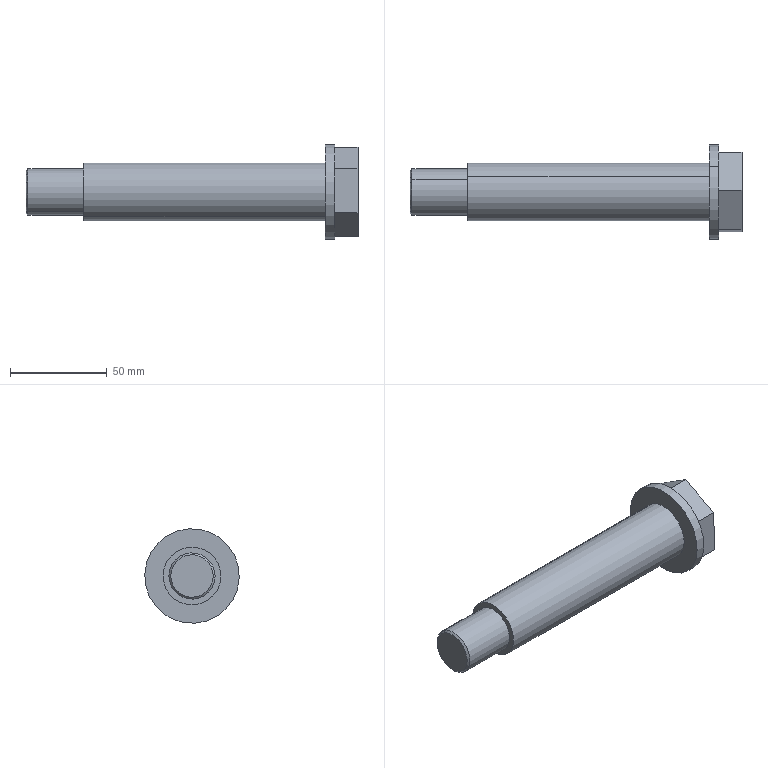Component | SolidWorks | SeedingAssemblyA-1_SeedingAxis-1 | 1 solid | 19 faces | box 172 x 49 x 49 mm | volume 127949 mm3 | plane 11 | cylinder 6 | cone 2 | commonest cylinder face diameters 24 x2 49 x2 30 x2
STEP:
#1=COLOUR_RGB('',0.7922,0.8196,0.9333);
#2=FILL_AREA_STYLE_COLOUR('',#1);
#3=FILL_AREA_STYLE('',(#2));
#4=SURFACE_STYLE_FILL_AREA(#3);
#5=SURFACE_SIDE_STYLE('',(#4));
#6=SURFACE_STYLE_USAGE(.BOTH.,#5);
#7=PRESENTATION_STYLE_ASSIGNMENT((#6));
#8=CARTESIAN_POINT('',(-0.3631,-3.902,-9.563));
#9=VERTEX_POINT('',#8);
#10=CARTESIAN_POINT('',(-0.3631,-4.366,-10.294));
#11=VERTEX_POINT('',#10);
#12=CARTESIAN_POINT('',(-0.3631,-4.134,-9.928));
#13=DIRECTION('',(-1.,0.,0.));
#14=DIRECTION('',(0.,0.5362,0.8441));
#15=AXIS2_PLACEMENT_3D('',#12,#13,#14);
#16=CIRCLE('',#15,0.4331);
#17=EDGE_CURVE('',#9,#11,#16,.T.);
#18=ORIENTED_EDGE('',*,*,#17,.F.);
#19=CARTESIAN_POINT('',(-0.3238,-3.881,-9.53));
#20=VERTEX_POINT('',#19);
#21=CARTESIAN_POINT('',(-0.3631,-3.902,-9.563));
#22=DIRECTION('',(0.7071,0.3792,0.5969));
#23=VECTOR('',#22,39.37);
#24=LINE('',#21,#23);
#25=EDGE_CURVE('',#9,#20,#24,.T.);
#26=ORIENTED_EDGE('',*,*,#25,.T.);
#27=CARTESIAN_POINT('',(-0.3238,-4.387,-10.327));
#28=VERTEX_POINT('',#27);
#29=CARTESIAN_POINT('',(-0.3238,-4.134,-9.928));
#30=DIRECTION('',(1.,-0.,-0.));
#31=DIRECTION('',(0.,0.5362,0.8441));
#32=AXIS2_PLACEMENT_3D('',#29,#30,#31);
#33=CIRCLE('',#32,0.4724);
#34=EDGE_CURVE('',#28,#20,#33,.T.);
#35=ORIENTED_EDGE('',*,*,#34,.F.);
#36=CARTESIAN_POINT('',(-0.3631,-4.366,-10.294));
#37=DIRECTION('',(0.7071,-0.3792,-0.5969));
#38=VECTOR('',#37,39.37);
#39=LINE('',#36,#38);
#40=EDGE_CURVE('',#11,#28,#39,.T.);
#41=ORIENTED_EDGE('',*,*,#40,.F.);
#42=EDGE_LOOP('',(#18,#26,#35,#41));
#43=FACE_OUTER_BOUND('',#42,.T.);
#44=CARTESIAN_POINT('',(-0.3631,-4.134,-9.928));
#45=DIRECTION('',(1.,-0.,-0.));
#46=DIRECTION('',(0.,-0.5362,-0.8441));
#47=AXIS2_PLACEMENT_3D('',#44,#45,#46);
#48=CONICAL_SURFACE('',#47,0.4331,0.7854);
#49=ADVANCED_FACE('',(#43),#48,.T.);
#50=ORIENTED_EDGE('',*,*,#34,.T.);
#51=CARTESIAN_POINT('',(0.818,-3.881,-9.53));
#52=VERTEX_POINT('',#51);
#53=CARTESIAN_POINT('',(-0.3631,-3.881,-9.53));
#54=DIRECTION('',(1.,-0.,-0.));
#55=VECTOR('',#54,39.37);
#56=LINE('',#53,#55);
#57=EDGE_CURVE('',#20,#52,#56,.T.);
#58=ORIENTED_EDGE('',*,*,#57,.T.);
#59=CARTESIAN_POINT('',(0.818,-4.387,-10.327));
#60=VERTEX_POINT('',#59);
#61=CARTESIAN_POINT('',(0.818,-4.134,-9.928));
#62=DIRECTION('',(-1.,0.,0.));
#63=DIRECTION('',(0.,0.5362,0.8441));
#64=AXIS2_PLACEMENT_3D('',#61,#62,#63);
#65=CIRCLE('',#64,0.4724);
#66=EDGE_CURVE('',#52,#60,#65,.T.);
#67=ORIENTED_EDGE('',*,*,#66,.T.);
#68=CARTESIAN_POINT('',(-0.3631,-4.387,-10.327));
#69=DIRECTION('',(1.,-0.,-0.));
#70=VECTOR('',#69,39.37);
#71=LINE('',#68,#70);
#72=EDGE_CURVE('',#28,#60,#71,.T.);
#73=ORIENTED_EDGE('',*,*,#72,.F.);
#74=EDGE_LOOP('',(#50,#58,#67,#73));
#75=FACE_OUTER_BOUND('',#74,.T.);
#76=CARTESIAN_POINT('',(-0.3631,-4.134,-9.928));
#77=DIRECTION('',(1.,-0.,-0.));
#78=DIRECTION('',(0.,-0.5362,-0.8441));
#79=AXIS2_PLACEMENT_3D('',#76,#77,#78);
#80=CYLINDRICAL_SURFACE('',#79,0.4724);
#81=ADVANCED_FACE('',(#75),#80,.T.);
#82=CARTESIAN_POINT('',(5.739,-3.617,-9.114));
#83=VERTEX_POINT('',#82);
#84=CARTESIAN_POINT('',(5.739,-4.651,-10.743));
#85=VERTEX_POINT('',#84);
#86=CARTESIAN_POINT('',(5.739,-4.134,-9.928));
#87=DIRECTION('',(-1.,0.,0.));
#88=DIRECTION('',(0.,0.5362,0.8441));
#89=AXIS2_PLACEMENT_3D('',#86,#87,#88);
#90=CIRCLE('',#89,0.9646);
#91=EDGE_CURVE('',#83,#85,#90,.T.);
#92=ORIENTED_EDGE('',*,*,#91,.F.);
#93=CARTESIAN_POINT('',(5.936,-3.617,-9.114));
#94=VERTEX_POINT('',#93);
#95=CARTESIAN_POINT('',(5.739,-3.617,-9.114));
#96=DIRECTION('',(1.,-0.,-0.));
#97=VECTOR('',#96,39.37);
#98=LINE('',#95,#97);
#99=EDGE_CURVE('',#83,#94,#98,.T.);
#100=ORIENTED_EDGE('',*,*,#99,.T.);
#101=CARTESIAN_POINT('',(5.936,-4.651,-10.743));
#102=VERTEX_POINT('',#101);
#103=CARTESIAN_POINT('',(5.936,-4.134,-9.928));
#104=DIRECTION('',(-1.,0.,0.));
#105=DIRECTION('',(0.,0.5362,0.8441));
#106=AXIS2_PLACEMENT_3D('',#103,#104,#105);
#107=CIRCLE('',#106,0.9646);
#108=EDGE_CURVE('',#94,#102,#107,.T.);
#109=ORIENTED_EDGE('',*,*,#108,.T.);
#110=CARTESIAN_POINT('',(5.739,-4.651,-10.743));
#111=DIRECTION('',(1.,-0.,-0.));
#112=VECTOR('',#111,39.37);
#113=LINE('',#110,#112);
#114=EDGE_CURVE('',#85,#102,#113,.T.);
#115=ORIENTED_EDGE('',*,*,#114,.F.);
#116=EDGE_LOOP('',(#92,#100,#109,#115));
#117=FACE_OUTER_BOUND('',#116,.T.);
#118=CARTESIAN_POINT('',(5.739,-4.134,-9.928));
#119=DIRECTION('',(1.,-0.,-0.));
#120=DIRECTION('',(0.,-0.5362,-0.8441));
#121=AXIS2_PLACEMENT_3D('',#118,#119,#120);
#122=CYLINDRICAL_SURFACE('',#121,0.9646);
#123=ADVANCED_FACE('',(#117),#122,.T.);
#124=CARTESIAN_POINT('',(0.818,-3.817,-9.43));
#125=VERTEX_POINT('',#124);
#126=CARTESIAN_POINT('',(0.818,-4.451,-10.427));
#127=VERTEX_POINT('',#126);
#128=CARTESIAN_POINT('',(0.818,-4.134,-9.928));
#129=DIRECTION('',(-1.,0.,0.));
#130=DIRECTION('',(0.,0.5362,0.8441));
#131=AXIS2_PLACEMENT_3D('',#128,#129,#130);
#132=CIRCLE('',#131,0.5906);
#133=EDGE_CURVE('',#125,#127,#132,.T.);
#134=ORIENTED_EDGE('',*,*,#133,.F.);
#135=CARTESIAN_POINT('',(5.739,-3.817,-9.43));
#136=VERTEX_POINT('',#135);
#137=CARTESIAN_POINT('',(0.818,-3.817,-9.43));
#138=DIRECTION('',(1.,-0.,-0.));
#139=VECTOR('',#138,39.37);
#140=LINE('',#137,#139);
#141=EDGE_CURVE('',#125,#136,#140,.T.);
#142=ORIENTED_EDGE('',*,*,#141,.T.);
#143=CARTESIAN_POINT('',(5.739,-4.451,-10.427));
#144=VERTEX_POINT('',#143);
#145=CARTESIAN_POINT('',(5.739,-4.134,-9.928));
#146=DIRECTION('',(-1.,0.,0.));
#147=DIRECTION('',(0.,0.5362,0.8441));
#148=AXIS2_PLACEMENT_3D('',#145,#146,#147);
#149=CIRCLE('',#148,0.5906);
#150=EDGE_CURVE('',#136,#144,#149,.T.);
#151=ORIENTED_EDGE('',*,*,#150,.T.);
#152=CARTESIAN_POINT('',(0.818,-4.451,-10.427));
#153=DIRECTION('',(1.,-0.,-0.));
#154=VECTOR('',#153,39.37);
#155=LINE('',#152,#154);
#156=EDGE_CURVE('',#127,#144,#155,.T.);
#157=ORIENTED_EDGE('',*,*,#156,.F.);
#158=EDGE_LOOP('',(#134,#142,#151,#157));
#159=FACE_OUTER_BOUND('',#158,.T.);
#160=CARTESIAN_POINT('',(0.818,-4.134,-9.928));
#161=DIRECTION('',(1.,-0.,-0.));
#162=DIRECTION('',(0.,-0.5362,-0.8441));
#163=AXIS2_PLACEMENT_3D('',#160,#161,#162);
#164=CYLINDRICAL_SURFACE('',#163,0.5906);
#165=ADVANCED_FACE('',(#159),#164,.T.);
#166=ORIENTED_EDGE('',*,*,#141,.F.);
#167=CARTESIAN_POINT('',(0.818,-4.134,-9.928));
#168=DIRECTION('',(-1.,0.,0.));
#169=DIRECTION('',(0.,0.5362,0.8441));
#170=AXIS2_PLACEMENT_3D('',#167,#168,#169);
#171=CIRCLE('',#170,0.5906);
#172=EDGE_CURVE('',#127,#125,#171,.T.);
#173=ORIENTED_EDGE('',*,*,#172,.F.);
#174=ORIENTED_EDGE('',*,*,#156,.T.);
#175=CARTESIAN_POINT('',(5.739,-4.134,-9.928));
#176=DIRECTION('',(-1.,0.,0.));
#177=DIRECTION('',(0.,0.5362,0.8441));
#178=AXIS2_PLACEMENT_3D('',#175,#176,#177);
#179=CIRCLE('',#178,0.5906);
#180=EDGE_CURVE('',#144,#136,#179,.T.);
#181=ORIENTED_EDGE('',*,*,#180,.T.);
#182=EDGE_LOOP('',(#166,#173,#174,#181));
#183=FACE_OUTER_BOUND('',#182,.T.);
#184=CARTESIAN_POINT('',(0.818,-4.134,-9.928));
#185=DIRECTION('',(1.,-0.,-0.));
#186=DIRECTION('',(0.,-0.5362,-0.8441));
#187=AXIS2_PLACEMENT_3D('',#184,#185,#186);
#188=CYLINDRICAL_SURFACE('',#187,0.5906);
#189=ADVANCED_FACE('',(#183),#188,.T.);
#190=CARTESIAN_POINT('',(0.818,-4.134,-9.928));
#191=DIRECTION('',(-1.,0.,0.));
#192=DIRECTION('',(0.,0.5362,0.8441));
#193=AXIS2_PLACEMENT_3D('',#190,#191,#192);
#194=CIRCLE('',#193,0.4724);
#195=EDGE_CURVE('',#60,#52,#194,.T.);
#196=ORIENTED_EDGE('',*,*,#195,.F.);
#197=ORIENTED_EDGE('',*,*,#66,.F.);
#198=EDGE_LOOP('',(#196,#197));
#199=FACE_BOUND('',#198,.T.);
#200=ORIENTED_EDGE('',*,*,#172,.T.);
#201=ORIENTED_EDGE('',*,*,#133,.T.);
#202=EDGE_LOOP('',(#200,#201));
#203=FACE_OUTER_BOUND('',#202,.T.);
#204=CARTESIAN_POINT('',(0.818,-4.134,-9.928));
#205=DIRECTION('',(-1.,0.,0.));
#206=DIRECTION('',(0.,0.5362,0.8441));
#207=AXIS2_PLACEMENT_3D('',#204,#205,#206);
#208=PLANE('',#207);
#209=ADVANCED_FACE('',(#199,#203),#208,.T.);
#210=CARTESIAN_POINT('',(5.936,-4.134,-9.928));
#211=DIRECTION('',(-1.,0.,0.));
#212=DIRECTION('',(0.,0.5362,0.8441));
#213=AXIS2_PLACEMENT_3D('',#210,#211,#212);
#214=CIRCLE('',#213,0.9646);
#215=EDGE_CURVE('',#102,#94,#214,.T.);
#216=ORIENTED_EDGE('',*,*,#215,.F.);
#217=ORIENTED_EDGE('',*,*,#108,.F.);
#218=EDGE_LOOP('',(#216,#217));
#219=FACE_OUTER_BOUND('',#218,.T.);
#220=CARTESIAN_POINT('',(5.936,-4.172,-10.837));
#221=VERTEX_POINT('',#220);
#222=CARTESIAN_POINT('',(5.936,-3.366,-10.416));
#223=VERTEX_POINT('',#222);
#224=CARTESIAN_POINT('',(5.936,-4.172,-10.837));
#225=DIRECTION('',(0.,0.8864,0.4629));
#226=VECTOR('',#225,39.37);
#227=LINE('',#224,#226);
#228=EDGE_CURVE('',#221,#223,#227,.T.);
#229=ORIENTED_EDGE('',*,*,#228,.F.);
#230=CARTESIAN_POINT('',(5.936,-4.94,-10.349));
#231=VERTEX_POINT('',#230);
#232=CARTESIAN_POINT('',(5.936,-4.94,-10.349));
#233=DIRECTION('',(0.,0.8441,-0.5362));
#234=VECTOR('',#233,39.37);
#235=LINE('',#232,#234);
#236=EDGE_CURVE('',#231,#221,#235,.T.);
#237=ORIENTED_EDGE('',*,*,#236,.F.);
#238=CARTESIAN_POINT('',(5.936,-4.901,-9.441));
#239=VERTEX_POINT('',#238);
#240=CARTESIAN_POINT('',(5.936,-4.901,-9.441));
#241=DIRECTION('',(-0.,-0.04234,-0.9991));
#242=VECTOR('',#241,39.37);
#243=LINE('',#240,#242);
#244=EDGE_CURVE('',#239,#231,#243,.T.);
#245=ORIENTED_EDGE('',*,*,#244,.F.);
#246=CARTESIAN_POINT('',(5.936,-4.095,-9.02));
#247=VERTEX_POINT('',#246);
#248=CARTESIAN_POINT('',(5.936,-4.095,-9.02));
#249=DIRECTION('',(-0.,-0.8864,-0.4629));
#250=VECTOR('',#249,39.37);
#251=LINE('',#248,#250);
#252=EDGE_CURVE('',#247,#239,#251,.T.);
#253=ORIENTED_EDGE('',*,*,#252,.F.);
#254=CARTESIAN_POINT('',(5.936,-3.328,-9.508));
#255=VERTEX_POINT('',#254);
#256=CARTESIAN_POINT('',(5.936,-3.328,-9.508));
#257=DIRECTION('',(-0.,-0.8441,0.5362));
#258=VECTOR('',#257,39.37);
#259=LINE('',#256,#258);
#260=EDGE_CURVE('',#255,#247,#259,.T.);
#261=ORIENTED_EDGE('',*,*,#260,.F.);
#262=CARTESIAN_POINT('',(5.936,-3.366,-10.416));
#263=DIRECTION('',(0.,0.04234,0.9991));
#264=VECTOR('',#263,39.37);
#265=LINE('',#262,#264);
#266=EDGE_CURVE('',#223,#255,#265,.T.);
#267=ORIENTED_EDGE('',*,*,#266,.F.);
#268=EDGE_LOOP('',(#229,#237,#245,#253,#261,#267));
#269=FACE_BOUND('',#268,.T.);
#270=CARTESIAN_POINT('',(5.936,-4.134,-9.928));
#271=DIRECTION('',(-1.,0.,0.));
#272=DIRECTION('',(0.,0.5362,0.8441));
#273=AXIS2_PLACEMENT_3D('',#270,#271,#272);
#274=PLANE('',#273);
#275=ADVANCED_FACE('',(#219,#269),#274,.F.);
#276=ORIENTED_EDGE('',*,*,#99,.F.);
#277=CARTESIAN_POINT('',(5.739,-4.134,-9.928));
#278=DIRECTION('',(-1.,0.,0.));
#279=DIRECTION('',(0.,0.5362,0.8441));
#280=AXIS2_PLACEMENT_3D('',#277,#278,#279);
#281=CIRCLE('',#280,0.9646);
#282=EDGE_CURVE('',#85,#83,#281,.T.);
#283=ORIENTED_EDGE('',*,*,#282,.F.);
#284=ORIENTED_EDGE('',*,*,#114,.T.);
#285=ORIENTED_EDGE('',*,*,#215,.T.);
#286=EDGE_LOOP('',(#276,#283,#284,#285));
#287=FACE_OUTER_BOUND('',#286,.T.);
#288=CARTESIAN_POINT('',(5.739,-4.134,-9.928));
#289=DIRECTION('',(1.,-0.,-0.));
#290=DIRECTION('',(0.,-0.5362,-0.8441));
#291=AXIS2_PLACEMENT_3D('',#288,#289,#290);
#292=CYLINDRICAL_SURFACE('',#291,0.9646);
#293=ADVANCED_FACE('',(#287),#292,.T.);
#294=ORIENTED_EDGE('',*,*,#180,.F.);
#295=ORIENTED_EDGE('',*,*,#150,.F.);
#296=EDGE_LOOP('',(#294,#295));
#297=FACE_BOUND('',#296,.T.);
#298=ORIENTED_EDGE('',*,*,#282,.T.);
#299=ORIENTED_EDGE('',*,*,#91,.T.);
#300=EDGE_LOOP('',(#298,#299));
#301=FACE_OUTER_BOUND('',#300,.T.);
#302=CARTESIAN_POINT('',(5.739,-4.134,-9.928));
#303=DIRECTION('',(-1.,0.,0.));
#304=DIRECTION('',(0.,0.5362,0.8441));
#305=AXIS2_PLACEMENT_3D('',#302,#303,#304);
#306=PLANE('',#305);
#307=ADVANCED_FACE('',(#297,#301),#306,.T.);
#308=CARTESIAN_POINT('',(6.409,-4.94,-10.349));
#309=VERTEX_POINT('',#308);
#310=CARTESIAN_POINT('',(6.409,-4.172,-10.837));
#311=VERTEX_POINT('',#310);
#312=CARTESIAN_POINT('',(6.409,-4.94,-10.349));
#313=DIRECTION('',(0.,0.8441,-0.5362));
#314=VECTOR('',#313,39.37);
#315=LINE('',#312,#314);
#316=EDGE_CURVE('',#309,#311,#315,.T.);
#317=ORIENTED_EDGE('',*,*,#316,.T.);
#318=CARTESIAN_POINT('',(6.409,-3.366,-10.416));
#319=VERTEX_POINT('',#318);
#320=CARTESIAN_POINT('',(6.409,-4.172,-10.837));
#321=DIRECTION('',(0.,0.8864,0.4629));
#322=VECTOR('',#321,39.37);
#323=LINE('',#320,#322);
#324=EDGE_CURVE('',#311,#319,#323,.T.);
#325=ORIENTED_EDGE('',*,*,#324,.T.);
#326=CARTESIAN_POINT('',(6.409,-3.328,-9.508));
#327=VERTEX_POINT('',#326);
#328=CARTESIAN_POINT('',(6.409,-3.366,-10.416));
#329=DIRECTION('',(0.,0.04234,0.9991));
#330=VECTOR('',#329,39.37);
#331=LINE('',#328,#330);
#332=EDGE_CURVE('',#319,#327,#331,.T.);
#333=ORIENTED_EDGE('',*,*,#332,.T.);
#334=CARTESIAN_POINT('',(6.409,-4.095,-9.02));
#335=VERTEX_POINT('',#334);
#336=CARTESIAN_POINT('',(6.409,-3.328,-9.508));
#337=DIRECTION('',(-0.,-0.8441,0.5362));
#338=VECTOR('',#337,39.37);
#339=LINE('',#336,#338);
#340=EDGE_CURVE('',#327,#335,#339,.T.);
#341=ORIENTED_EDGE('',*,*,#340,.T.);
#342=CARTESIAN_POINT('',(6.409,-4.901,-9.441));
#343=VERTEX_POINT('',#342);
#344=CARTESIAN_POINT('',(6.409,-4.095,-9.02));
#345=DIRECTION('',(-0.,-0.8864,-0.4629));
#346=VECTOR('',#345,39.37);
#347=LINE('',#344,#346);
#348=EDGE_CURVE('',#335,#343,#347,.T.);
#349=ORIENTED_EDGE('',*,*,#348,.T.);
#350=CARTESIAN_POINT('',(6.409,-4.901,-9.441));
#351=DIRECTION('',(-0.,-0.04234,-0.9991));
#352=VECTOR('',#351,39.37);
#353=LINE('',#350,#352);
#354=EDGE_CURVE('',#343,#309,#353,.T.);
#355=ORIENTED_EDGE('',*,*,#354,.T.);
#356=EDGE_LOOP('',(#317,#325,#333,#341,#349,#355));
#357=FACE_OUTER_BOUND('',#356,.T.);
#358=CARTESIAN_POINT('',(6.409,-4.134,-9.928));
#359=DIRECTION('',(1.,-0.,-0.));
#360=DIRECTION('',(-0.,-0.5362,-0.8441));
#361=AXIS2_PLACEMENT_3D('',#358,#359,#360);
#362=PLANE('',#361);
#363=ADVANCED_FACE('',(#357),#362,.T.);
#364=ORIENTED_EDGE('',*,*,#244,.T.);
#365=CARTESIAN_POINT('',(6.409,-4.94,-10.349));
#366=DIRECTION('',(-1.,0.,0.));
#367=VECTOR('',#366,39.37);
#368=LINE('',#365,#367);
#369=EDGE_CURVE('',#309,#231,#368,.T.);
#370=ORIENTED_EDGE('',*,*,#369,.F.);
#371=ORIENTED_EDGE('',*,*,#354,.F.);
#372=CARTESIAN_POINT('',(6.409,-4.901,-9.441));
#373=DIRECTION('',(-1.,0.,0.));
#374=VECTOR('',#373,39.37);
#375=LINE('',#372,#374);
#376=EDGE_CURVE('',#343,#239,#375,.T.);
#377=ORIENTED_EDGE('',*,*,#376,.T.);
#378=EDGE_LOOP('',(#364,#370,#371,#377));
#379=FACE_OUTER_BOUND('',#378,.T.);
#380=CARTESIAN_POINT('',(6.409,-4.901,-9.441));
#381=DIRECTION('',(0.,0.9991,-0.04234));
#382=DIRECTION('',(-0.,-0.04234,-0.9991));
#383=AXIS2_PLACEMENT_3D('',#380,#381,#382);
#384=PLANE('',#383);
#385=ADVANCED_FACE('',(#379),#384,.F.);
#386=ORIENTED_EDGE('',*,*,#252,.T.);
#387=ORIENTED_EDGE('',*,*,#376,.F.);
#388=ORIENTED_EDGE('',*,*,#348,.F.);
#389=CARTESIAN_POINT('',(6.409,-4.095,-9.02));
#390=DIRECTION('',(-1.,0.,0.));
#391=VECTOR('',#390,39.37);
#392=LINE('',#389,#391);
#393=EDGE_CURVE('',#335,#247,#392,.T.);
#394=ORIENTED_EDGE('',*,*,#393,.T.);
#395=EDGE_LOOP('',(#386,#387,#388,#394));
#396=FACE_OUTER_BOUND('',#395,.T.);
#397=CARTESIAN_POINT('',(6.409,-4.095,-9.02));
#398=DIRECTION('',(-0.,0.4629,-0.8864));
#399=DIRECTION('',(-0.,-0.8864,-0.4629));
#400=AXIS2_PLACEMENT_3D('',#397,#398,#399);
#401=PLANE('',#400);
#402=ADVANCED_FACE('',(#396),#401,.F.);
#403=ORIENTED_EDGE('',*,*,#260,.T.);
#404=ORIENTED_EDGE('',*,*,#393,.F.);
#405=ORIENTED_EDGE('',*,*,#340,.F.);
#406=CARTESIAN_POINT('',(6.409,-3.328,-9.508));
#407=DIRECTION('',(-1.,0.,0.));
#408=VECTOR('',#407,39.37);
#409=LINE('',#406,#408);
#410=EDGE_CURVE('',#327,#255,#409,.T.);
#411=ORIENTED_EDGE('',*,*,#410,.T.);
#412=EDGE_LOOP('',(#403,#404,#405,#411));
#413=FACE_OUTER_BOUND('',#412,.T.);
#414=CARTESIAN_POINT('',(6.409,-3.328,-9.508));
#415=DIRECTION('',(-0.,-0.5362,-0.8441));
#416=DIRECTION('',(-0.,-0.8441,0.5362));
#417=AXIS2_PLACEMENT_3D('',#414,#415,#416);
#418=PLANE('',#417);
#419=ADVANCED_FACE('',(#413),#418,.F.);
#420=ORIENTED_EDGE('',*,*,#266,.T.);
#421=ORIENTED_EDGE('',*,*,#410,.F.);
#422=ORIENTED_EDGE('',*,*,#332,.F.);
#423=CARTESIAN_POINT('',(6.409,-3.366,-10.416));
#424=DIRECTION('',(-1.,0.,0.));
#425=VECTOR('',#424,39.37);
#426=LINE('',#423,#425);
#427=EDGE_CURVE('',#319,#223,#426,.T.);
#428=ORIENTED_EDGE('',*,*,#427,.T.);
#429=EDGE_LOOP('',(#420,#421,#422,#428));
#430=FACE_OUTER_BOUND('',#429,.T.);
#431=CARTESIAN_POINT('',(6.409,-3.366,-10.416));
#432=DIRECTION('',(-0.,-0.9991,0.04234));
#433=DIRECTION('',(0.,0.04234,0.9991));
#434=AXIS2_PLACEMENT_3D('',#431,#432,#433);
#435=PLANE('',#434);
#436=ADVANCED_FACE('',(#430),#435,.F.);
#437=ORIENTED_EDGE('',*,*,#228,.T.);
#438=ORIENTED_EDGE('',*,*,#427,.F.);
#439=ORIENTED_EDGE('',*,*,#324,.F.);
#440=CARTESIAN_POINT('',(6.409,-4.172,-10.837));
#441=DIRECTION('',(-1.,0.,0.));
#442=VECTOR('',#441,39.37);
#443=LINE('',#440,#442);
#444=EDGE_CURVE('',#311,#221,#443,.T.);
#445=ORIENTED_EDGE('',*,*,#444,.T.);
#446=EDGE_LOOP('',(#437,#438,#439,#445));
#447=FACE_OUTER_BOUND('',#446,.T.);
#448=CARTESIAN_POINT('',(6.409,-4.172,-10.837));
#449=DIRECTION('',(0.,-0.4629,0.8864));
#450=DIRECTION('',(0.,0.8864,0.4629));
#451=AXIS2_PLACEMENT_3D('',#448,#449,#450);
#452=PLANE('',#451);
#453=ADVANCED_FACE('',(#447),#452,.F.);
#454=ORIENTED_EDGE('',*,*,#236,.T.);
#455=ORIENTED_EDGE('',*,*,#444,.F.);
#456=ORIENTED_EDGE('',*,*,#316,.F.);
#457=ORIENTED_EDGE('',*,*,#369,.T.);
#458=EDGE_LOOP('',(#454,#455,#456,#457));
#459=FACE_OUTER_BOUND('',#458,.T.);
#460=CARTESIAN_POINT('',(6.409,-4.94,-10.349));
#461=DIRECTION('',(0.,0.5362,0.8441));
#462=DIRECTION('',(0.,0.8441,-0.5362));
#463=AXIS2_PLACEMENT_3D('',#460,#461,#462);
#464=PLANE('',#463);
#465=ADVANCED_FACE('',(#459),#464,.F.);
#466=ORIENTED_EDGE('',*,*,#57,.F.);
#467=CARTESIAN_POINT('',(-0.3238,-4.134,-9.928));
#468=DIRECTION('',(1.,-0.,-0.));
#469=DIRECTION('',(0.,0.5362,0.8441));
#470=AXIS2_PLACEMENT_3D('',#467,#468,#469);
#471=CIRCLE('',#470,0.4724);
#472=EDGE_CURVE('',#20,#28,#471,.T.);
#473=ORIENTED_EDGE('',*,*,#472,.T.);
#474=ORIENTED_EDGE('',*,*,#72,.T.);
#475=ORIENTED_EDGE('',*,*,#195,.T.);
#476=EDGE_LOOP('',(#466,#473,#474,#475));
#477=FACE_OUTER_BOUND('',#476,.T.);
#478=CARTESIAN_POINT('',(-0.3631,-4.134,-9.928));
#479=DIRECTION('',(1.,-0.,-0.));
#480=DIRECTION('',(0.,-0.5362,-0.8441));
#481=AXIS2_PLACEMENT_3D('',#478,#479,#480);
#482=CYLINDRICAL_SURFACE('',#481,0.4724);
#483=ADVANCED_FACE('',(#477),#482,.T.);
#484=CARTESIAN_POINT('',(-0.3631,-4.134,-9.928));
#485=DIRECTION('',(-1.,0.,0.));
#486=DIRECTION('',(0.,0.5362,0.8441));
#487=AXIS2_PLACEMENT_3D('',#484,#485,#486);
#488=CIRCLE('',#487,0.4331);
#489=EDGE_CURVE('',#11,#9,#488,.T.);
#490=ORIENTED_EDGE('',*,*,#489,.T.);
#491=ORIENTED_EDGE('',*,*,#17,.T.);
#492=EDGE_LOOP('',(#490,#491));
#493=FACE_OUTER_BOUND('',#492,.T.);
#494=CARTESIAN_POINT('',(-0.3631,-4.134,-9.928));
#495=DIRECTION('',(-1.,0.,0.));
#496=DIRECTION('',(0.,0.5362,0.8441));
#497=AXIS2_PLACEMENT_3D('',#494,#495,#496);
#498=PLANE('',#497);
#499=ADVANCED_FACE('',(#493),#498,.T.);
#500=ORIENTED_EDGE('',*,*,#25,.F.);
#501=ORIENTED_EDGE('',*,*,#489,.F.);
#502=ORIENTED_EDGE('',*,*,#40,.T.);
#503=ORIENTED_EDGE('',*,*,#472,.F.);
#504=EDGE_LOOP('',(#500,#501,#502,#503));
#505=FACE_OUTER_BOUND('',#504,.T.);
#506=CARTESIAN_POINT('',(-0.3631,-4.134,-9.928));
#507=DIRECTION('',(1.,-0.,-0.));
#508=DIRECTION('',(0.,-0.5362,-0.8441));
#509=AXIS2_PLACEMENT_3D('',#506,#507,#508);
#510=CONICAL_SURFACE('',#509,0.4331,0.7854);
#511=ADVANCED_FACE('',(#505),#510,.T.);
#512=CLOSED_SHELL('',(#49,#81,#123,#165,#189,#209,#275,#293,#307,#363,#385,#402,#419,#436,#453,#465,#483,#499,#511));
#513=MANIFOLD_SOLID_BREP('',#512);
#514=STYLED_ITEM('',(#7),#513);
#515=(LENGTH_UNIT()NAMED_UNIT(*)SI_UNIT($,.METRE.));
#516=LENGTH_MEASURE_WITH_UNIT(LENGTH_MEASURE(0.0254),#515);
#517=DIMENSIONAL_EXPONENTS(1.,0.,0.,0.,0.,0.,0.);
#518=(CONVERSION_BASED_UNIT('',#516)LENGTH_UNIT()NAMED_UNIT(#517));
#519=UNCERTAINTY_MEASURE_WITH_UNIT(LENGTH_MEASURE(0.00001),#518,'','');
#520=(NAMED_UNIT(*)PLANE_ANGLE_UNIT()SI_UNIT($,.RADIAN.));
#521=(NAMED_UNIT(*)SI_UNIT($,.STERADIAN.)SOLID_ANGLE_UNIT());
#522=(GEOMETRIC_REPRESENTATION_CONTEXT(3)GLOBAL_UNCERTAINTY_ASSIGNED_CONTEXT((#519))GLOBAL_UNIT_ASSIGNED_CONTEXT((#518,#520,#521))REPRESENTATION_CONTEXT('',''));
#523=MECHANICAL_DESIGN_GEOMETRIC_PRESENTATION_REPRESENTATION('',(#514),#522);
#524=PRESENTATION_LAYER_ASSIGNMENT('','',(#514));
#525=CARTESIAN_POINT('',(0.,0.,0.));
#526=DIRECTION('',(0.,0.,1.));
#527=DIRECTION('',(1.,0.,0.));
#528=AXIS2_PLACEMENT_3D('',#525,#526,#527);
#529=(LENGTH_UNIT()NAMED_UNIT(*)SI_UNIT($,.METRE.));
#530=LENGTH_MEASURE_WITH_UNIT(LENGTH_MEASURE(0.0254),#529);
#531=DIMENSIONAL_EXPONENTS(1.,0.,0.,0.,0.,0.,0.);
#532=(CONVERSION_BASED_UNIT('',#530)LENGTH_UNIT()NAMED_UNIT(#531));
#533=UNCERTAINTY_MEASURE_WITH_UNIT(LENGTH_MEASURE(0.00001),#532,'','');
#534=(NAMED_UNIT(*)PLANE_ANGLE_UNIT()SI_UNIT($,.RADIAN.));
#535=(NAMED_UNIT(*)SI_UNIT($,.STERADIAN.)SOLID_ANGLE_UNIT());
#536=(GEOMETRIC_REPRESENTATION_CONTEXT(3)GLOBAL_UNCERTAINTY_ASSIGNED_CONTEXT((#533))GLOBAL_UNIT_ASSIGNED_CONTEXT((#532,#534,#535))REPRESENTATION_CONTEXT('',''));
#537=ADVANCED_BREP_SHAPE_REPRESENTATION('',(#513,#528),#536);